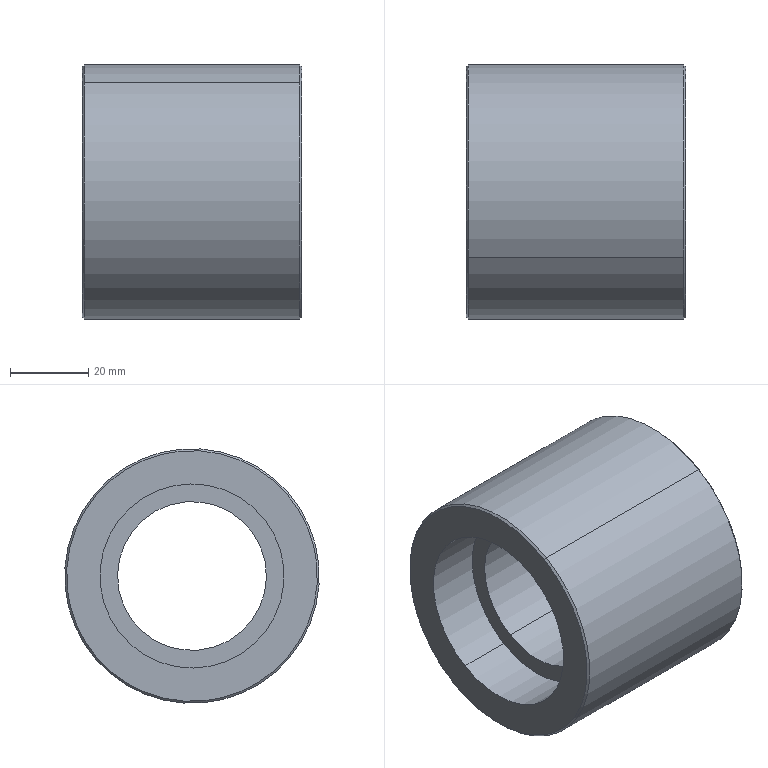Component | SolidWorks | PressHeadBearingHousing-1 | 1 solid | 36 faces | box 56 x 65 x 65 mm | volume 103574 mm3 | cylinder 20 | plane 10 | cone 6 | commonest cylinder face diameters 4.2 x12 47 x4 65 x2 38 x2
STEP:
#1=COLOUR_RGB('',0.7922,0.8196,0.9333);
#2=FILL_AREA_STYLE_COLOUR('',#1);
#3=FILL_AREA_STYLE('',(#2));
#4=SURFACE_STYLE_FILL_AREA(#3);
#5=SURFACE_SIDE_STYLE('',(#4));
#6=SURFACE_STYLE_USAGE(.BOTH.,#5);
#7=PRESENTATION_STYLE_ASSIGNMENT((#6));
#8=CARTESIAN_POINT('',(16.809,50.693,27.845));
#9=VERTEX_POINT('',#8);
#10=CARTESIAN_POINT('',(16.809,51.646,26.259));
#11=VERTEX_POINT('',#10);
#12=CARTESIAN_POINT('',(16.809,51.17,27.052));
#13=DIRECTION('',(-1.,-0.,-0.));
#14=DIRECTION('',(-0.,0.515,-0.8572));
#15=AXIS2_PLACEMENT_3D('',#12,#13,#14);
#16=CIRCLE('',#15,0.9252);
#17=EDGE_CURVE('',#9,#11,#16,.T.);
#18=ORIENTED_EDGE('',*,*,#17,.F.);
#19=CARTESIAN_POINT('',(16.257,50.693,27.845));
#20=VERTEX_POINT('',#19);
#21=CARTESIAN_POINT('',(16.809,50.693,27.845));
#22=DIRECTION('',(-1.,-0.,-0.));
#23=VECTOR('',#22,39.37);
#24=LINE('',#21,#23);
#25=EDGE_CURVE('',#9,#20,#24,.T.);
#26=ORIENTED_EDGE('',*,*,#25,.T.);
#27=CARTESIAN_POINT('',(16.257,51.646,26.259));
#28=VERTEX_POINT('',#27);
#29=CARTESIAN_POINT('',(16.257,51.17,27.052));
#30=DIRECTION('',(-1.,-0.,-0.));
#31=DIRECTION('',(-0.,0.515,-0.8572));
#32=AXIS2_PLACEMENT_3D('',#29,#30,#31);
#33=CIRCLE('',#32,0.9252);
#34=EDGE_CURVE('',#20,#28,#33,.T.);
#35=ORIENTED_EDGE('',*,*,#34,.T.);
#36=CARTESIAN_POINT('',(16.809,51.646,26.259));
#37=DIRECTION('',(-1.,-0.,-0.));
#38=VECTOR('',#37,39.37);
#39=LINE('',#36,#38);
#40=EDGE_CURVE('',#11,#28,#39,.T.);
#41=ORIENTED_EDGE('',*,*,#40,.F.);
#42=EDGE_LOOP('',(#18,#26,#35,#41));
#43=FACE_OUTER_BOUND('',#42,.T.);
#44=CARTESIAN_POINT('',(16.809,51.17,27.052));
#45=DIRECTION('',(-1.,-0.,-0.));
#46=DIRECTION('',(-0.,0.515,-0.8572));
#47=AXIS2_PLACEMENT_3D('',#44,#45,#46);
#48=CYLINDRICAL_SURFACE('',#47,0.9252);
#49=ADVANCED_FACE('',(#43),#48,.F.);
#50=CARTESIAN_POINT('',(17.872,51.231,25.879));
#51=VERTEX_POINT('',#50);
#52=CARTESIAN_POINT('',(17.872,51.146,26.02));
#53=VERTEX_POINT('',#52);
#54=CARTESIAN_POINT('',(17.872,51.189,25.95));
#55=DIRECTION('',(1.,0.,0.));
#56=DIRECTION('',(0.,-0.515,0.8572));
#57=AXIS2_PLACEMENT_3D('',#54,#55,#56);
#58=CIRCLE('',#57,0.08268);
#59=EDGE_CURVE('',#51,#53,#58,.T.);
#60=ORIENTED_EDGE('',*,*,#59,.F.);
#61=CARTESIAN_POINT('',(18.462,51.231,25.879));
#62=VERTEX_POINT('',#61);
#63=CARTESIAN_POINT('',(17.872,51.231,25.879));
#64=DIRECTION('',(1.,0.,0.));
#65=VECTOR('',#64,39.37);
#66=LINE('',#63,#65);
#67=EDGE_CURVE('',#51,#62,#66,.T.);
#68=ORIENTED_EDGE('',*,*,#67,.T.);
#69=CARTESIAN_POINT('',(18.462,51.146,26.02));
#70=VERTEX_POINT('',#69);
#71=CARTESIAN_POINT('',(18.462,51.189,25.95));
#72=DIRECTION('',(1.,0.,0.));
#73=DIRECTION('',(0.,-0.515,0.8572));
#74=AXIS2_PLACEMENT_3D('',#71,#72,#73);
#75=CIRCLE('',#74,0.08268);
#76=EDGE_CURVE('',#62,#70,#75,.T.);
#77=ORIENTED_EDGE('',*,*,#76,.T.);
#78=CARTESIAN_POINT('',(17.872,51.146,26.02));
#79=DIRECTION('',(1.,0.,0.));
#80=VECTOR('',#79,39.37);
#81=LINE('',#78,#80);
#82=EDGE_CURVE('',#53,#70,#81,.T.);
#83=ORIENTED_EDGE('',*,*,#82,.F.);
#84=EDGE_LOOP('',(#60,#68,#77,#83));
#85=FACE_OUTER_BOUND('',#84,.T.);
#86=CARTESIAN_POINT('',(17.872,51.189,25.95));
#87=DIRECTION('',(1.,0.,0.));
#88=DIRECTION('',(0.,-0.515,0.8572));
#89=AXIS2_PLACEMENT_3D('',#86,#87,#88);
#90=CYLINDRICAL_SURFACE('',#89,0.08268);
#91=ADVANCED_FACE('',(#85),#90,.F.);
#92=CARTESIAN_POINT('',(17.872,52.176,26.447));
#93=VERTEX_POINT('',#92);
#94=CARTESIAN_POINT('',(17.872,52.091,26.588));
#95=VERTEX_POINT('',#94);
#96=CARTESIAN_POINT('',(17.872,52.134,26.517));
#97=DIRECTION('',(1.,0.,0.));
#98=DIRECTION('',(0.,-0.515,0.8572));
#99=AXIS2_PLACEMENT_3D('',#96,#97,#98);
#100=CIRCLE('',#99,0.08268);
#101=EDGE_CURVE('',#93,#95,#100,.T.);
#102=ORIENTED_EDGE('',*,*,#101,.F.);
#103=CARTESIAN_POINT('',(18.462,52.176,26.447));
#104=VERTEX_POINT('',#103);
#105=CARTESIAN_POINT('',(17.872,52.176,26.447));
#106=DIRECTION('',(1.,0.,0.));
#107=VECTOR('',#106,39.37);
#108=LINE('',#105,#107);
#109=EDGE_CURVE('',#93,#104,#108,.T.);
#110=ORIENTED_EDGE('',*,*,#109,.T.);
#111=CARTESIAN_POINT('',(18.462,52.091,26.588));
#112=VERTEX_POINT('',#111);
#113=CARTESIAN_POINT('',(18.462,52.134,26.517));
#114=DIRECTION('',(1.,0.,0.));
#115=DIRECTION('',(0.,-0.515,0.8572));
#116=AXIS2_PLACEMENT_3D('',#113,#114,#115);
#117=CIRCLE('',#116,0.08268);
#118=EDGE_CURVE('',#104,#112,#117,.T.);
#119=ORIENTED_EDGE('',*,*,#118,.T.);
#120=CARTESIAN_POINT('',(17.872,52.091,26.588));
#121=DIRECTION('',(1.,0.,0.));
#122=VECTOR('',#121,39.37);
#123=LINE('',#120,#122);
#124=EDGE_CURVE('',#95,#112,#123,.T.);
#125=ORIENTED_EDGE('',*,*,#124,.F.);
#126=EDGE_LOOP('',(#102,#110,#119,#125));
#127=FACE_OUTER_BOUND('',#126,.T.);
#128=CARTESIAN_POINT('',(17.872,52.134,26.517));
#129=DIRECTION('',(1.,0.,0.));
#130=DIRECTION('',(0.,-0.515,0.8572));
#131=AXIS2_PLACEMENT_3D('',#128,#129,#130);
#132=CYLINDRICAL_SURFACE('',#131,0.08268);
#133=ADVANCED_FACE('',(#127),#132,.F.);
#134=CARTESIAN_POINT('',(17.872,52.157,27.549));
#135=VERTEX_POINT('',#134);
#136=CARTESIAN_POINT('',(17.872,52.072,27.69));
#137=VERTEX_POINT('',#136);
#138=CARTESIAN_POINT('',(17.872,52.114,27.62));
#139=DIRECTION('',(1.,0.,0.));
#140=DIRECTION('',(0.,-0.515,0.8572));
#141=AXIS2_PLACEMENT_3D('',#138,#139,#140);
#142=CIRCLE('',#141,0.08268);
#143=EDGE_CURVE('',#135,#137,#142,.T.);
#144=ORIENTED_EDGE('',*,*,#143,.F.);
#145=CARTESIAN_POINT('',(18.462,52.157,27.549));
#146=VERTEX_POINT('',#145);
#147=CARTESIAN_POINT('',(17.872,52.157,27.549));
#148=DIRECTION('',(1.,0.,0.));
#149=VECTOR('',#148,39.37);
#150=LINE('',#147,#149);
#151=EDGE_CURVE('',#135,#146,#150,.T.);
#152=ORIENTED_EDGE('',*,*,#151,.T.);
#153=CARTESIAN_POINT('',(18.462,52.072,27.69));
#154=VERTEX_POINT('',#153);
#155=CARTESIAN_POINT('',(18.462,52.114,27.62));
#156=DIRECTION('',(1.,0.,0.));
#157=DIRECTION('',(0.,-0.515,0.8572));
#158=AXIS2_PLACEMENT_3D('',#155,#156,#157);
#159=CIRCLE('',#158,0.08268);
#160=EDGE_CURVE('',#146,#154,#159,.T.);
#161=ORIENTED_EDGE('',*,*,#160,.T.);
#162=CARTESIAN_POINT('',(17.872,52.072,27.69));
#163=DIRECTION('',(1.,0.,0.));
#164=VECTOR('',#163,39.37);
#165=LINE('',#162,#164);
#166=EDGE_CURVE('',#137,#154,#165,.T.);
#167=ORIENTED_EDGE('',*,*,#166,.F.);
#168=EDGE_LOOP('',(#144,#152,#161,#167));
#169=FACE_OUTER_BOUND('',#168,.T.);
#170=CARTESIAN_POINT('',(17.872,52.114,27.62));
#171=DIRECTION('',(1.,0.,0.));
#172=DIRECTION('',(0.,-0.515,0.8572));
#173=AXIS2_PLACEMENT_3D('',#170,#171,#172);
#174=CYLINDRICAL_SURFACE('',#173,0.08268);
#175=ADVANCED_FACE('',(#169),#174,.F.);
#176=CARTESIAN_POINT('',(17.872,51.193,28.083));
#177=VERTEX_POINT('',#176);
#178=CARTESIAN_POINT('',(17.872,51.108,28.225));
#179=VERTEX_POINT('',#178);
#180=CARTESIAN_POINT('',(17.872,51.15,28.154));
#181=DIRECTION('',(1.,0.,0.));
#182=DIRECTION('',(0.,-0.515,0.8572));
#183=AXIS2_PLACEMENT_3D('',#180,#181,#182);
#184=CIRCLE('',#183,0.08268);
#185=EDGE_CURVE('',#177,#179,#184,.T.);
#186=ORIENTED_EDGE('',*,*,#185,.F.);
#187=CARTESIAN_POINT('',(18.462,51.193,28.083));
#188=VERTEX_POINT('',#187);
#189=CARTESIAN_POINT('',(17.872,51.193,28.083));
#190=DIRECTION('',(1.,0.,0.));
#191=VECTOR('',#190,39.37);
#192=LINE('',#189,#191);
#193=EDGE_CURVE('',#177,#188,#192,.T.);
#194=ORIENTED_EDGE('',*,*,#193,.T.);
#195=CARTESIAN_POINT('',(18.462,51.108,28.225));
#196=VERTEX_POINT('',#195);
#197=CARTESIAN_POINT('',(18.462,51.15,28.154));
#198=DIRECTION('',(1.,0.,0.));
#199=DIRECTION('',(0.,-0.515,0.8572));
#200=AXIS2_PLACEMENT_3D('',#197,#198,#199);
#201=CIRCLE('',#200,0.08268);
#202=EDGE_CURVE('',#188,#196,#201,.T.);
#203=ORIENTED_EDGE('',*,*,#202,.T.);
#204=CARTESIAN_POINT('',(17.872,51.108,28.225));
#205=DIRECTION('',(1.,0.,0.));
#206=VECTOR('',#205,39.37);
#207=LINE('',#204,#206);
#208=EDGE_CURVE('',#179,#196,#207,.T.);
#209=ORIENTED_EDGE('',*,*,#208,.F.);
#210=EDGE_LOOP('',(#186,#194,#203,#209));
#211=FACE_OUTER_BOUND('',#210,.T.);
#212=CARTESIAN_POINT('',(17.872,51.15,28.154));
#213=DIRECTION('',(1.,0.,0.));
#214=DIRECTION('',(0.,-0.515,0.8572));
#215=AXIS2_PLACEMENT_3D('',#212,#213,#214);
#216=CYLINDRICAL_SURFACE('',#215,0.08268);
#217=ADVANCED_FACE('',(#211),#216,.F.);
#218=CARTESIAN_POINT('',(17.872,50.267,26.413));
#219=VERTEX_POINT('',#218);
#220=CARTESIAN_POINT('',(17.872,50.182,26.555));
#221=VERTEX_POINT('',#220);
#222=CARTESIAN_POINT('',(17.872,50.225,26.484));
#223=DIRECTION('',(1.,0.,0.));
#224=DIRECTION('',(0.,-0.515,0.8572));
#225=AXIS2_PLACEMENT_3D('',#222,#223,#224);
#226=CIRCLE('',#225,0.08268);
#227=EDGE_CURVE('',#219,#221,#226,.T.);
#228=ORIENTED_EDGE('',*,*,#227,.F.);
#229=CARTESIAN_POINT('',(18.462,50.267,26.413));
#230=VERTEX_POINT('',#229);
#231=CARTESIAN_POINT('',(17.872,50.267,26.413));
#232=DIRECTION('',(1.,0.,0.));
#233=VECTOR('',#232,39.37);
#234=LINE('',#231,#233);
#235=EDGE_CURVE('',#219,#230,#234,.T.);
#236=ORIENTED_EDGE('',*,*,#235,.T.);
#237=CARTESIAN_POINT('',(18.462,50.182,26.555));
#238=VERTEX_POINT('',#237);
#239=CARTESIAN_POINT('',(18.462,50.225,26.484));
#240=DIRECTION('',(1.,0.,0.));
#241=DIRECTION('',(0.,-0.515,0.8572));
#242=AXIS2_PLACEMENT_3D('',#239,#240,#241);
#243=CIRCLE('',#242,0.08268);
#244=EDGE_CURVE('',#230,#238,#243,.T.);
#245=ORIENTED_EDGE('',*,*,#244,.T.);
#246=CARTESIAN_POINT('',(17.872,50.182,26.555));
#247=DIRECTION('',(1.,0.,0.));
#248=VECTOR('',#247,39.37);
#249=LINE('',#246,#248);
#250=EDGE_CURVE('',#221,#238,#249,.T.);
#251=ORIENTED_EDGE('',*,*,#250,.F.);
#252=EDGE_LOOP('',(#228,#236,#245,#251));
#253=FACE_OUTER_BOUND('',#252,.T.);
#254=CARTESIAN_POINT('',(17.872,50.225,26.484));
#255=DIRECTION('',(1.,0.,0.));
#256=DIRECTION('',(0.,-0.515,0.8572));
#257=AXIS2_PLACEMENT_3D('',#254,#255,#256);
#258=CYLINDRICAL_SURFACE('',#257,0.08268);
#259=ADVANCED_FACE('',(#253),#258,.F.);
#260=CARTESIAN_POINT('',(17.872,50.248,27.515));
#261=VERTEX_POINT('',#260);
#262=CARTESIAN_POINT('',(17.872,50.163,27.657));
#263=VERTEX_POINT('',#262);
#264=CARTESIAN_POINT('',(17.872,50.205,27.586));
#265=DIRECTION('',(1.,0.,0.));
#266=DIRECTION('',(0.,-0.515,0.8572));
#267=AXIS2_PLACEMENT_3D('',#264,#265,#266);
#268=CIRCLE('',#267,0.08268);
#269=EDGE_CURVE('',#261,#263,#268,.T.);
#270=ORIENTED_EDGE('',*,*,#269,.F.);
#271=CARTESIAN_POINT('',(18.462,50.248,27.515));
#272=VERTEX_POINT('',#271);
#273=CARTESIAN_POINT('',(17.872,50.248,27.515));
#274=DIRECTION('',(1.,0.,0.));
#275=VECTOR('',#274,39.37);
#276=LINE('',#273,#275);
#277=EDGE_CURVE('',#261,#272,#276,.T.);
#278=ORIENTED_EDGE('',*,*,#277,.T.);
#279=CARTESIAN_POINT('',(18.462,50.163,27.657));
#280=VERTEX_POINT('',#279);
#281=CARTESIAN_POINT('',(18.462,50.205,27.586));
#282=DIRECTION('',(1.,0.,0.));
#283=DIRECTION('',(0.,-0.515,0.8572));
#284=AXIS2_PLACEMENT_3D('',#281,#282,#283);
#285=CIRCLE('',#284,0.08268);
#286=EDGE_CURVE('',#272,#280,#285,.T.);
#287=ORIENTED_EDGE('',*,*,#286,.T.);
#288=CARTESIAN_POINT('',(17.872,50.163,27.657));
#289=DIRECTION('',(1.,0.,0.));
#290=VECTOR('',#289,39.37);
#291=LINE('',#288,#290);
#292=EDGE_CURVE('',#263,#280,#291,.T.);
#293=ORIENTED_EDGE('',*,*,#292,.F.);
#294=EDGE_LOOP('',(#270,#278,#287,#293));
#295=FACE_OUTER_BOUND('',#294,.T.);
#296=CARTESIAN_POINT('',(17.872,50.205,27.586));
#297=DIRECTION('',(1.,0.,0.));
#298=DIRECTION('',(0.,-0.515,0.8572));
#299=AXIS2_PLACEMENT_3D('',#296,#297,#298);
#300=CYLINDRICAL_SURFACE('',#299,0.08268);
#301=ADVANCED_FACE('',(#295),#300,.F.);
#302=CARTESIAN_POINT('',(18.442,51.646,26.259));
#303=VERTEX_POINT('',#302);
#304=CARTESIAN_POINT('',(18.442,50.693,27.845));
#305=VERTEX_POINT('',#304);
#306=CARTESIAN_POINT('',(18.442,51.17,27.052));
#307=DIRECTION('',(1.,0.,0.));
#308=DIRECTION('',(0.,-0.515,0.8572));
#309=AXIS2_PLACEMENT_3D('',#306,#307,#308);
#310=CIRCLE('',#309,0.9252);
#311=EDGE_CURVE('',#303,#305,#310,.T.);
#312=ORIENTED_EDGE('',*,*,#311,.F.);
#313=CARTESIAN_POINT('',(18.462,51.656,26.242));
#314=VERTEX_POINT('',#313);
#315=CARTESIAN_POINT('',(18.442,51.646,26.259));
#316=DIRECTION('',(0.7071,0.3642,-0.6061));
#317=VECTOR('',#316,39.37);
#318=LINE('',#315,#317);
#319=EDGE_CURVE('',#303,#314,#318,.T.);
#320=ORIENTED_EDGE('',*,*,#319,.T.);
#321=CARTESIAN_POINT('',(18.462,50.683,27.862));
#322=VERTEX_POINT('',#321);
#323=CARTESIAN_POINT('',(18.462,51.17,27.052));
#324=DIRECTION('',(-1.,-0.,-0.));
#325=DIRECTION('',(0.,-0.515,0.8572));
#326=AXIS2_PLACEMENT_3D('',#323,#324,#325);
#327=CIRCLE('',#326,0.9449);
#328=EDGE_CURVE('',#322,#314,#327,.T.);
#329=ORIENTED_EDGE('',*,*,#328,.F.);
#330=CARTESIAN_POINT('',(18.442,50.693,27.845));
#331=DIRECTION('',(0.7071,-0.3642,0.6061));
#332=VECTOR('',#331,39.37);
#333=LINE('',#330,#332);
#334=EDGE_CURVE('',#305,#322,#333,.T.);
#335=ORIENTED_EDGE('',*,*,#334,.F.);
#336=EDGE_LOOP('',(#312,#320,#329,#335));
#337=FACE_OUTER_BOUND('',#336,.T.);
#338=CARTESIAN_POINT('',(18.442,51.17,27.052));
#339=DIRECTION('',(1.,0.,0.));
#340=DIRECTION('',(0.,-0.515,0.8572));
#341=AXIS2_PLACEMENT_3D('',#338,#339,#340);
#342=CONICAL_SURFACE('',#341,0.9252,0.7854);
#343=ADVANCED_FACE('',(#337),#342,.F.);
#344=CARTESIAN_POINT('',(18.462,50.521,28.132));
#345=VERTEX_POINT('',#344);
#346=CARTESIAN_POINT('',(18.462,51.818,25.972));
#347=VERTEX_POINT('',#346);
#348=CARTESIAN_POINT('',(18.462,51.17,27.052));
#349=DIRECTION('',(1.,0.,0.));
#350=DIRECTION('',(0.,-0.515,0.8572));
#351=AXIS2_PLACEMENT_3D('',#348,#349,#350);
#352=CIRCLE('',#351,1.26);
#353=EDGE_CURVE('',#345,#347,#352,.T.);
#354=ORIENTED_EDGE('',*,*,#353,.F.);
#355=CARTESIAN_POINT('',(18.442,50.511,28.149));
#356=VERTEX_POINT('',#355);
#357=CARTESIAN_POINT('',(18.462,50.521,28.132));
#358=DIRECTION('',(-0.7071,-0.3642,0.6061));
#359=VECTOR('',#358,39.37);
#360=LINE('',#357,#359);
#361=EDGE_CURVE('',#345,#356,#360,.T.);
#362=ORIENTED_EDGE('',*,*,#361,.T.);
#363=CARTESIAN_POINT('',(18.442,51.829,25.955));
#364=VERTEX_POINT('',#363);
#365=CARTESIAN_POINT('',(18.442,51.17,27.052));
#366=DIRECTION('',(-1.,-0.,-0.));
#367=DIRECTION('',(0.,-0.515,0.8572));
#368=AXIS2_PLACEMENT_3D('',#365,#366,#367);
#369=CIRCLE('',#368,1.28);
#370=EDGE_CURVE('',#364,#356,#369,.T.);
#371=ORIENTED_EDGE('',*,*,#370,.F.);
#372=CARTESIAN_POINT('',(18.462,51.818,25.972));
#373=DIRECTION('',(-0.7071,0.3642,-0.6061));
#374=VECTOR('',#373,39.37);
#375=LINE('',#372,#374);
#376=EDGE_CURVE('',#347,#364,#375,.T.);
#377=ORIENTED_EDGE('',*,*,#376,.F.);
#378=EDGE_LOOP('',(#354,#362,#371,#377));
#379=FACE_OUTER_BOUND('',#378,.T.);
#380=CARTESIAN_POINT('',(18.462,51.17,27.052));
#381=DIRECTION('',(-1.,-0.,-0.));
#382=DIRECTION('',(-0.,0.515,-0.8572));
#383=AXIS2_PLACEMENT_3D('',#380,#381,#382);
#384=CONICAL_SURFACE('',#383,1.26,0.7854);
#385=ADVANCED_FACE('',(#379),#384,.T.);
#386=CARTESIAN_POINT('',(16.257,51.818,25.972));
#387=VERTEX_POINT('',#386);
#388=CARTESIAN_POINT('',(16.257,50.521,28.132));
#389=VERTEX_POINT('',#388);
#390=CARTESIAN_POINT('',(16.257,51.17,27.052));
#391=DIRECTION('',(-1.,-0.,-0.));
#392=DIRECTION('',(0.,-0.515,0.8572));
#393=AXIS2_PLACEMENT_3D('',#390,#391,#392);
#394=CIRCLE('',#393,1.26);
#395=EDGE_CURVE('',#387,#389,#394,.T.);
#396=ORIENTED_EDGE('',*,*,#395,.F.);
#397=CARTESIAN_POINT('',(16.277,51.829,25.955));
#398=VERTEX_POINT('',#397);
#399=CARTESIAN_POINT('',(16.277,51.829,25.955));
#400=DIRECTION('',(0.7071,0.3642,-0.6061));
#401=VECTOR('',#400,39.37);
#402=LINE('',#399,#401);
#403=EDGE_CURVE('',#387,#398,#402,.T.);
#404=ORIENTED_EDGE('',*,*,#403,.T.);
#405=CARTESIAN_POINT('',(16.277,50.511,28.149));
#406=VERTEX_POINT('',#405);
#407=CARTESIAN_POINT('',(16.277,51.17,27.052));
#408=DIRECTION('',(1.,0.,0.));
#409=DIRECTION('',(0.,-0.515,0.8572));
#410=AXIS2_PLACEMENT_3D('',#407,#408,#409);
#411=CIRCLE('',#410,1.28);
#412=EDGE_CURVE('',#406,#398,#411,.T.);
#413=ORIENTED_EDGE('',*,*,#412,.F.);
#414=CARTESIAN_POINT('',(16.277,50.511,28.149));
#415=DIRECTION('',(0.7071,-0.3642,0.6061));
#416=VECTOR('',#415,39.37);
#417=LINE('',#414,#416);
#418=EDGE_CURVE('',#389,#406,#417,.T.);
#419=ORIENTED_EDGE('',*,*,#418,.F.);
#420=EDGE_LOOP('',(#396,#404,#413,#419));
#421=FACE_OUTER_BOUND('',#420,.T.);
#422=CARTESIAN_POINT('',(16.277,51.17,27.052));
#423=DIRECTION('',(1.,0.,0.));
#424=DIRECTION('',(0.,-0.515,0.8572));
#425=AXIS2_PLACEMENT_3D('',#422,#423,#424);
#426=CONICAL_SURFACE('',#425,1.28,0.7854);
#427=ADVANCED_FACE('',(#421),#426,.T.);
#428=CARTESIAN_POINT('',(17.872,51.646,26.259));
#429=VERTEX_POINT('',#428);
#430=CARTESIAN_POINT('',(17.872,50.693,27.845));
#431=VERTEX_POINT('',#430);
#432=CARTESIAN_POINT('',(17.872,51.17,27.052));
#433=DIRECTION('',(1.,0.,0.));
#434=DIRECTION('',(0.,-0.515,0.8572));
#435=AXIS2_PLACEMENT_3D('',#432,#433,#434);
#436=CIRCLE('',#435,0.9252);
#437=EDGE_CURVE('',#429,#431,#436,.T.);
#438=ORIENTED_EDGE('',*,*,#437,.F.);
#439=CARTESIAN_POINT('',(17.872,51.646,26.259));
#440=DIRECTION('',(1.,0.,0.));
#441=VECTOR('',#440,39.37);
#442=LINE('',#439,#441);
#443=EDGE_CURVE('',#429,#303,#442,.T.);
#444=ORIENTED_EDGE('',*,*,#443,.T.);
#445=ORIENTED_EDGE('',*,*,#311,.T.);
#446=CARTESIAN_POINT('',(17.872,50.693,27.845));
#447=DIRECTION('',(1.,0.,0.));
#448=VECTOR('',#447,39.37);
#449=LINE('',#446,#448);
#450=EDGE_CURVE('',#431,#305,#449,.T.);
#451=ORIENTED_EDGE('',*,*,#450,.F.);
#452=EDGE_LOOP('',(#438,#444,#445,#451));
#453=FACE_OUTER_BOUND('',#452,.T.);
#454=CARTESIAN_POINT('',(17.872,51.17,27.052));
#455=DIRECTION('',(1.,0.,0.));
#456=DIRECTION('',(0.,-0.515,0.8572));
#457=AXIS2_PLACEMENT_3D('',#454,#455,#456);
#458=CYLINDRICAL_SURFACE('',#457,0.9252);
#459=ADVANCED_FACE('',(#453),#458,.F.);
#460=ORIENTED_EDGE('',*,*,#370,.T.);
#461=CARTESIAN_POINT('',(17.045,50.511,28.149));
#462=DIRECTION('',(-1.,-0.,-0.));
#463=VECTOR('',#462,39.37);
#464=LINE('',#461,#463);
#465=EDGE_CURVE('',#356,#406,#464,.T.);
#466=ORIENTED_EDGE('',*,*,#465,.T.);
#467=ORIENTED_EDGE('',*,*,#412,.T.);
#468=CARTESIAN_POINT('',(17.045,51.829,25.955));
#469=DIRECTION('',(-1.,-0.,-0.));
#470=VECTOR('',#469,39.37);
#471=LINE('',#468,#470);
#472=EDGE_CURVE('',#364,#398,#471,.T.);
#473=ORIENTED_EDGE('',*,*,#472,.F.);
#474=EDGE_LOOP('',(#460,#466,#467,#473));
#475=FACE_OUTER_BOUND('',#474,.T.);
#476=CARTESIAN_POINT('',(17.045,51.17,27.052));
#477=DIRECTION('',(-1.,-0.,-0.));
#478=DIRECTION('',(-0.,0.515,-0.8572));
#479=AXIS2_PLACEMENT_3D('',#476,#477,#478);
#480=CYLINDRICAL_SURFACE('',#479,1.28);
#481=ADVANCED_FACE('',(#475),#480,.T.);
#482=CARTESIAN_POINT('',(16.809,51.555,26.411));
#483=VERTEX_POINT('',#482);
#484=CARTESIAN_POINT('',(16.809,50.784,27.693));
#485=VERTEX_POINT('',#484);
#486=CARTESIAN_POINT('',(16.809,51.17,27.052));
#487=DIRECTION('',(1.,0.,0.));
#488=DIRECTION('',(-0.,0.515,-0.8572));
#489=AXIS2_PLACEMENT_3D('',#486,#487,#488);
#490=CIRCLE('',#489,0.748);
#491=EDGE_CURVE('',#483,#485,#490,.T.);
#492=ORIENTED_EDGE('',*,*,#491,.F.);
#493=CARTESIAN_POINT('',(17.872,51.555,26.411));
#494=VERTEX_POINT('',#493);
#495=CARTESIAN_POINT('',(16.257,51.555,26.411));
#496=DIRECTION('',(1.,0.,0.));
#497=VECTOR('',#496,39.37);
#498=LINE('',#495,#497);
#499=EDGE_CURVE('',#483,#494,#498,.T.);
#500=ORIENTED_EDGE('',*,*,#499,.T.);
#501=CARTESIAN_POINT('',(17.872,50.784,27.693));
#502=VERTEX_POINT('',#501);
#503=CARTESIAN_POINT('',(17.872,51.17,27.052));
#504=DIRECTION('',(1.,0.,0.));
#505=DIRECTION('',(0.,-0.515,0.8572));
#506=AXIS2_PLACEMENT_3D('',#503,#504,#505);
#507=CIRCLE('',#506,0.748);
#508=EDGE_CURVE('',#494,#502,#507,.T.);
#509=ORIENTED_EDGE('',*,*,#508,.T.);
#510=CARTESIAN_POINT('',(16.257,50.784,27.693));
#511=DIRECTION('',(1.,0.,0.));
#512=VECTOR('',#511,39.37);
#513=LINE('',#510,#512);
#514=EDGE_CURVE('',#485,#502,#513,.T.);
#515=ORIENTED_EDGE('',*,*,#514,.F.);
#516=EDGE_LOOP('',(#492,#500,#509,#515));
#517=FACE_OUTER_BOUND('',#516,.T.);
#518=CARTESIAN_POINT('',(16.257,51.17,27.052));
#519=DIRECTION('',(1.,0.,0.));
#520=DIRECTION('',(0.,-0.515,0.8572));
#521=AXIS2_PLACEMENT_3D('',#518,#519,#520);
#522=CYLINDRICAL_SURFACE('',#521,0.748);
#523=ADVANCED_FACE('',(#517),#522,.F.);
#524=ORIENTED_EDGE('',*,*,#499,.F.);
#525=CARTESIAN_POINT('',(16.809,51.17,27.052));
#526=DIRECTION('',(1.,0.,0.));
#527=DIRECTION('',(-0.,0.515,-0.8572));
#528=AXIS2_PLACEMENT_3D('',#525,#526,#527);
#529=CIRCLE('',#528,0.748);
#530=EDGE_CURVE('',#485,#483,#529,.T.);
#531=ORIENTED_EDGE('',*,*,#530,.F.);
#532=ORIENTED_EDGE('',*,*,#514,.T.);
#533=CARTESIAN_POINT('',(17.872,51.17,27.052));
#534=DIRECTION('',(1.,0.,0.));
#535=DIRECTION('',(0.,-0.515,0.8572));
#536=AXIS2_PLACEMENT_3D('',#533,#534,#535);
#537=CIRCLE('',#536,0.748);
#538=EDGE_CURVE('',#502,#494,#537,.T.);
#539=ORIENTED_EDGE('',*,*,#538,.T.);
#540=EDGE_LOOP('',(#524,#531,#532,#539));
#541=FACE_OUTER_BOUND('',#540,.T.);
#542=CARTESIAN_POINT('',(16.257,51.17,27.052));
#543=DIRECTION('',(1.,0.,0.));
#544=DIRECTION('',(0.,-0.515,0.8572));
#545=AXIS2_PLACEMENT_3D('',#542,#543,#544);
#546=CYLINDRICAL_SURFACE('',#545,0.748);
#547=ADVANCED_FACE('',(#541),#546,.F.);
#548=ORIENTED_EDGE('',*,*,#465,.F.);
#549=CARTESIAN_POINT('',(18.442,51.17,27.052));
#550=DIRECTION('',(-1.,-0.,-0.));
#551=DIRECTION('',(0.,-0.515,0.8572));
#552=AXIS2_PLACEMENT_3D('',#549,#550,#551);
#553=CIRCLE('',#552,1.28);
#554=EDGE_CURVE('',#356,#364,#553,.T.);
#555=ORIENTED_EDGE('',*,*,#554,.T.);
#556=ORIENTED_EDGE('',*,*,#472,.T.);
#557=CARTESIAN_POINT('',(16.277,51.17,27.052));
#558=DIRECTION('',(1.,0.,0.));
#559=DIRECTION('',(0.,-0.515,0.8572));
#560=AXIS2_PLACEMENT_3D('',#557,#558,#559);
#561=CIRCLE('',#560,1.28);
#562=EDGE_CURVE('',#398,#406,#561,.T.);
#563=ORIENTED_EDGE('',*,*,#562,.T.);
#564=EDGE_LOOP('',(#548,#555,#556,#563));
#565=FACE_OUTER_BOUND('',#564,.T.);
#566=CARTESIAN_POINT('',(17.045,51.17,27.052));
#567=DIRECTION('',(-1.,-0.,-0.));
#568=DIRECTION('',(-0.,0.515,-0.8572));
#569=AXIS2_PLACEMENT_3D('',#566,#567,#568);
#570=CYLINDRICAL_SURFACE('',#569,1.28);
#571=ADVANCED_FACE('',(#565),#570,.T.);
#572=CARTESIAN_POINT('',(16.257,51.17,27.052));
#573=DIRECTION('',(-1.,-0.,-0.));
#574=DIRECTION('',(-0.,0.515,-0.8572));
#575=AXIS2_PLACEMENT_3D('',#572,#573,#574);
#576=CIRCLE('',#575,0.9252);
#577=EDGE_CURVE('',#28,#20,#576,.T.);
#578=ORIENTED_EDGE('',*,*,#577,.F.);
#579=ORIENTED_EDGE('',*,*,#34,.F.);
#580=EDGE_LOOP('',(#578,#579));
#581=FACE_BOUND('',#580,.T.);
#582=CARTESIAN_POINT('',(16.257,51.17,27.052));
#583=DIRECTION('',(-1.,-0.,-0.));
#584=DIRECTION('',(0.,-0.515,0.8572));
#585=AXIS2_PLACEMENT_3D('',#582,#583,#584);
#586=CIRCLE('',#585,1.26);
#587=EDGE_CURVE('',#389,#387,#586,.T.);
#588=ORIENTED_EDGE('',*,*,#587,.T.);
#589=ORIENTED_EDGE('',*,*,#395,.T.);
#590=EDGE_LOOP('',(#588,#589));
#591=FACE_OUTER_BOUND('',#590,.T.);
#592=CARTESIAN_POINT('',(16.257,51.17,27.052));
#593=DIRECTION('',(1.,0.,0.));
#594=DIRECTION('',(0.,-0.515,0.8572));
#595=AXIS2_PLACEMENT_3D('',#592,#593,#594);
#596=PLANE('',#595);
#597=ADVANCED_FACE('',(#581,#591),#596,.F.);
#598=CARTESIAN_POINT('',(18.462,51.189,25.95));
#599=DIRECTION('',(1.,0.,0.));
#600=DIRECTION('',(0.,-0.515,0.8572));
#601=AXIS2_PLACEMENT_3D('',#598,#599,#600);
#602=CIRCLE('',#601,0.08268);
#603=EDGE_CURVE('',#70,#62,#602,.T.);
#604=ORIENTED_EDGE('',*,*,#603,.F.);
#605=ORIENTED_EDGE('',*,*,#76,.F.);
#606=EDGE_LOOP('',(#604,#605));
#607=FACE_BOUND('',#606,.T.);
#608=CARTESIAN_POINT('',(18.462,52.134,26.517));
#609=DIRECTION('',(1.,0.,0.));
#610=DIRECTION('',(0.,-0.515,0.8572));
#611=AXIS2_PLACEMENT_3D('',#608,#609,#610);
#612=CIRCLE('',#611,0.08268);
#613=EDGE_CURVE('',#112,#104,#612,.T.);
#614=ORIENTED_EDGE('',*,*,#613,.F.);
#615=ORIENTED_EDGE('',*,*,#118,.F.);
#616=EDGE_LOOP('',(#614,#615));
#617=FACE_BOUND('',#616,.T.);
#618=CARTESIAN_POINT('',(18.462,52.114,27.62));
#619=DIRECTION('',(1.,0.,0.));
#620=DIRECTION('',(0.,-0.515,0.8572));
#621=AXIS2_PLACEMENT_3D('',#618,#619,#620);
#622=CIRCLE('',#621,0.08268);
#623=EDGE_CURVE('',#154,#146,#622,.T.);
#624=ORIENTED_EDGE('',*,*,#623,.F.);
#625=ORIENTED_EDGE('',*,*,#160,.F.);
#626=EDGE_LOOP('',(#624,#625));
#627=FACE_BOUND('',#626,.T.);
#628=CARTESIAN_POINT('',(18.462,51.15,28.154));
#629=DIRECTION('',(1.,0.,0.));
#630=DIRECTION('',(0.,-0.515,0.8572));
#631=AXIS2_PLACEMENT_3D('',#628,#629,#630);
#632=CIRCLE('',#631,0.08268);
#633=EDGE_CURVE('',#196,#188,#632,.T.);
#634=ORIENTED_EDGE('',*,*,#633,.F.);
#635=ORIENTED_EDGE('',*,*,#202,.F.);
#636=EDGE_LOOP('',(#634,#635));
#637=FACE_BOUND('',#636,.T.);
#638=CARTESIAN_POINT('',(18.462,50.225,26.484));
#639=DIRECTION('',(1.,0.,0.));
#640=DIRECTION('',(0.,-0.515,0.8572));
#641=AXIS2_PLACEMENT_3D('',#638,#639,#640);
#642=CIRCLE('',#641,0.08268);
#643=EDGE_CURVE('',#238,#230,#642,.T.);
#644=ORIENTED_EDGE('',*,*,#643,.F.);
#645=ORIENTED_EDGE('',*,*,#244,.F.);
#646=EDGE_LOOP('',(#644,#645));
#647=FACE_BOUND('',#646,.T.);
#648=CARTESIAN_POINT('',(18.462,50.205,27.586));
#649=DIRECTION('',(1.,0.,0.));
#650=DIRECTION('',(0.,-0.515,0.8572));
#651=AXIS2_PLACEMENT_3D('',#648,#649,#650);
#652=CIRCLE('',#651,0.08268);
#653=EDGE_CURVE('',#280,#272,#652,.T.);
#654=ORIENTED_EDGE('',*,*,#653,.F.);
#655=ORIENTED_EDGE('',*,*,#286,.F.);
#656=EDGE_LOOP('',(#654,#655));
#657=FACE_BOUND('',#656,.T.);
#658=CARTESIAN_POINT('',(18.462,51.17,27.052));
#659=DIRECTION('',(1.,0.,0.));
#660=DIRECTION('',(0.,-0.515,0.8572));
#661=AXIS2_PLACEMENT_3D('',#658,#659,#660);
#662=CIRCLE('',#661,1.26);
#663=EDGE_CURVE('',#347,#345,#662,.T.);
#664=ORIENTED_EDGE('',*,*,#663,.T.);
#665=ORIENTED_EDGE('',*,*,#353,.T.);
#666=EDGE_LOOP('',(#664,#665));
#667=FACE_OUTER_BOUND('',#666,.T.);
#668=ORIENTED_EDGE('',*,*,#328,.T.);
#669=CARTESIAN_POINT('',(18.462,51.17,27.052));
#670=DIRECTION('',(-1.,-0.,-0.));
#671=DIRECTION('',(0.,-0.515,0.8572));
#672=AXIS2_PLACEMENT_3D('',#669,#670,#671);
#673=CIRCLE('',#672,0.9449);
#674=EDGE_CURVE('',#314,#322,#673,.T.);
#675=ORIENTED_EDGE('',*,*,#674,.T.);
#676=EDGE_LOOP('',(#668,#675));
#677=FACE_BOUND('',#676,.T.);
#678=CARTESIAN_POINT('',(18.462,51.17,27.052));
#679=DIRECTION('',(1.,0.,0.));
#680=DIRECTION('',(0.,-0.515,0.8572));
#681=AXIS2_PLACEMENT_3D('',#678,#679,#680);
#682=PLANE('',#681);
#683=ADVANCED_FACE('',(#607,#617,#627,#637,#647,#657,#667,#677),#682,.T.);
#684=ORIENTED_EDGE('',*,*,#443,.F.);
#685=CARTESIAN_POINT('',(17.872,51.17,27.052));
#686=DIRECTION('',(1.,0.,0.));
#687=DIRECTION('',(0.,-0.515,0.8572));
#688=AXIS2_PLACEMENT_3D('',#685,#686,#687);
#689=CIRCLE('',#688,0.9252);
#690=EDGE_CURVE('',#431,#429,#689,.T.);
#691=ORIENTED_EDGE('',*,*,#690,.F.);
#692=ORIENTED_EDGE('',*,*,#450,.T.);
#693=CARTESIAN_POINT('',(18.442,51.17,27.052));
#694=DIRECTION('',(1.,0.,0.));
#695=DIRECTION('',(0.,-0.515,0.8572));
#696=AXIS2_PLACEMENT_3D('',#693,#694,#695);
#697=CIRCLE('',#696,0.9252);
#698=EDGE_CURVE('',#305,#303,#697,.T.);
#699=ORIENTED_EDGE('',*,*,#698,.T.);
#700=EDGE_LOOP('',(#684,#691,#692,#699));
#701=FACE_OUTER_BOUND('',#700,.T.);
#702=CARTESIAN_POINT('',(17.872,51.17,27.052));
#703=DIRECTION('',(1.,0.,0.));
#704=DIRECTION('',(0.,-0.515,0.8572));
#705=AXIS2_PLACEMENT_3D('',#702,#703,#704);
#706=CYLINDRICAL_SURFACE('',#705,0.9252);
#707=ADVANCED_FACE('',(#701),#706,.F.);
#708=ORIENTED_EDGE('',*,*,#538,.F.);
#709=ORIENTED_EDGE('',*,*,#508,.F.);
#710=EDGE_LOOP('',(#708,#709));
#711=FACE_BOUND('',#710,.T.);
#712=ORIENTED_EDGE('',*,*,#690,.T.);
#713=ORIENTED_EDGE('',*,*,#437,.T.);
#714=EDGE_LOOP('',(#712,#713));
#715=FACE_OUTER_BOUND('',#714,.T.);
#716=CARTESIAN_POINT('',(17.872,51.17,27.052));
#717=DIRECTION('',(1.,0.,0.));
#718=DIRECTION('',(0.,-0.515,0.8572));
#719=AXIS2_PLACEMENT_3D('',#716,#717,#718);
#720=PLANE('',#719);
#721=ADVANCED_FACE('',(#711,#715),#720,.T.);
#722=ORIENTED_EDGE('',*,*,#403,.F.);
#723=ORIENTED_EDGE('',*,*,#587,.F.);
#724=ORIENTED_EDGE('',*,*,#418,.T.);
#725=ORIENTED_EDGE('',*,*,#562,.F.);
#726=EDGE_LOOP('',(#722,#723,#724,#725));
#727=FACE_OUTER_BOUND('',#726,.T.);
#728=CARTESIAN_POINT('',(16.277,51.17,27.052));
#729=DIRECTION('',(1.,0.,0.));
#730=DIRECTION('',(0.,-0.515,0.8572));
#731=AXIS2_PLACEMENT_3D('',#728,#729,#730);
#732=CONICAL_SURFACE('',#731,1.28,0.7854);
#733=ADVANCED_FACE('',(#727),#732,.T.);
#734=ORIENTED_EDGE('',*,*,#361,.F.);
#735=ORIENTED_EDGE('',*,*,#663,.F.);
#736=ORIENTED_EDGE('',*,*,#376,.T.);
#737=ORIENTED_EDGE('',*,*,#554,.F.);
#738=EDGE_LOOP('',(#734,#735,#736,#737));
#739=FACE_OUTER_BOUND('',#738,.T.);
#740=CARTESIAN_POINT('',(18.462,51.17,27.052));
#741=DIRECTION('',(-1.,-0.,-0.));
#742=DIRECTION('',(-0.,0.515,-0.8572));
#743=AXIS2_PLACEMENT_3D('',#740,#741,#742);
#744=CONICAL_SURFACE('',#743,1.26,0.7854);
#745=ADVANCED_FACE('',(#739),#744,.T.);
#746=ORIENTED_EDGE('',*,*,#319,.F.);
#747=ORIENTED_EDGE('',*,*,#698,.F.);
#748=ORIENTED_EDGE('',*,*,#334,.T.);
#749=ORIENTED_EDGE('',*,*,#674,.F.);
#750=EDGE_LOOP('',(#746,#747,#748,#749));
#751=FACE_OUTER_BOUND('',#750,.T.);
#752=CARTESIAN_POINT('',(18.442,51.17,27.052));
#753=DIRECTION('',(1.,0.,0.));
#754=DIRECTION('',(0.,-0.515,0.8572));
#755=AXIS2_PLACEMENT_3D('',#752,#753,#754);
#756=CONICAL_SURFACE('',#755,0.9252,0.7854);
#757=ADVANCED_FACE('',(#751),#756,.F.);
#758=ORIENTED_EDGE('',*,*,#277,.F.);
#759=CARTESIAN_POINT('',(17.872,50.205,27.586));
#760=DIRECTION('',(1.,0.,0.));
#761=DIRECTION('',(0.,-0.515,0.8572));
#762=AXIS2_PLACEMENT_3D('',#759,#760,#761);
#763=CIRCLE('',#762,0.08268);
#764=EDGE_CURVE('',#263,#261,#763,.T.);
#765=ORIENTED_EDGE('',*,*,#764,.F.);
#766=ORIENTED_EDGE('',*,*,#292,.T.);
#767=ORIENTED_EDGE('',*,*,#653,.T.);
#768=EDGE_LOOP('',(#758,#765,#766,#767));
#769=FACE_OUTER_BOUND('',#768,.T.);
#770=CARTESIAN_POINT('',(17.872,50.205,27.586));
#771=DIRECTION('',(1.,0.,0.));
#772=DIRECTION('',(0.,-0.515,0.8572));
#773=AXIS2_PLACEMENT_3D('',#770,#771,#772);
#774=CYLINDRICAL_SURFACE('',#773,0.08268);
#775=ADVANCED_FACE('',(#769),#774,.F.);
#776=ORIENTED_EDGE('',*,*,#764,.T.);
#777=ORIENTED_EDGE('',*,*,#269,.T.);
#778=EDGE_LOOP('',(#776,#777));
#779=FACE_OUTER_BOUND('',#778,.T.);
#780=CARTESIAN_POINT('',(17.872,50.205,27.586));
#781=DIRECTION('',(1.,0.,0.));
#782=DIRECTION('',(0.,-0.515,0.8572));
#783=AXIS2_PLACEMENT_3D('',#780,#781,#782);
#784=PLANE('',#783);
#785=ADVANCED_FACE('',(#779),#784,.T.);
#786=ORIENTED_EDGE('',*,*,#235,.F.);
#787=CARTESIAN_POINT('',(17.872,50.225,26.484));
#788=DIRECTION('',(1.,0.,0.));
#789=DIRECTION('',(0.,-0.515,0.8572));
#790=AXIS2_PLACEMENT_3D('',#787,#788,#789);
#791=CIRCLE('',#790,0.08268);
#792=EDGE_CURVE('',#221,#219,#791,.T.);
#793=ORIENTED_EDGE('',*,*,#792,.F.);
#794=ORIENTED_EDGE('',*,*,#250,.T.);
#795=ORIENTED_EDGE('',*,*,#643,.T.);
#796=EDGE_LOOP('',(#786,#793,#794,#795));
#797=FACE_OUTER_BOUND('',#796,.T.);
#798=CARTESIAN_POINT('',(17.872,50.225,26.484));
#799=DIRECTION('',(1.,0.,0.));
#800=DIRECTION('',(0.,-0.515,0.8572));
#801=AXIS2_PLACEMENT_3D('',#798,#799,#800);
#802=CYLINDRICAL_SURFACE('',#801,0.08268);
#803=ADVANCED_FACE('',(#797),#802,.F.);
#804=ORIENTED_EDGE('',*,*,#792,.T.);
#805=ORIENTED_EDGE('',*,*,#227,.T.);
#806=EDGE_LOOP('',(#804,#805));
#807=FACE_OUTER_BOUND('',#806,.T.);
#808=CARTESIAN_POINT('',(17.872,50.225,26.484));
#809=DIRECTION('',(1.,0.,0.));
#810=DIRECTION('',(0.,-0.515,0.8572));
#811=AXIS2_PLACEMENT_3D('',#808,#809,#810);
#812=PLANE('',#811);
#813=ADVANCED_FACE('',(#807),#812,.T.);
#814=ORIENTED_EDGE('',*,*,#193,.F.);
#815=CARTESIAN_POINT('',(17.872,51.15,28.154));
#816=DIRECTION('',(1.,0.,0.));
#817=DIRECTION('',(0.,-0.515,0.8572));
#818=AXIS2_PLACEMENT_3D('',#815,#816,#817);
#819=CIRCLE('',#818,0.08268);
#820=EDGE_CURVE('',#179,#177,#819,.T.);
#821=ORIENTED_EDGE('',*,*,#820,.F.);
#822=ORIENTED_EDGE('',*,*,#208,.T.);
#823=ORIENTED_EDGE('',*,*,#633,.T.);
#824=EDGE_LOOP('',(#814,#821,#822,#823));
#825=FACE_OUTER_BOUND('',#824,.T.);
#826=CARTESIAN_POINT('',(17.872,51.15,28.154));
#827=DIRECTION('',(1.,0.,0.));
#828=DIRECTION('',(0.,-0.515,0.8572));
#829=AXIS2_PLACEMENT_3D('',#826,#827,#828);
#830=CYLINDRICAL_SURFACE('',#829,0.08268);
#831=ADVANCED_FACE('',(#825),#830,.F.);
#832=ORIENTED_EDGE('',*,*,#820,.T.);
#833=ORIENTED_EDGE('',*,*,#185,.T.);
#834=EDGE_LOOP('',(#832,#833));
#835=FACE_OUTER_BOUND('',#834,.T.);
#836=CARTESIAN_POINT('',(17.872,51.15,28.154));
#837=DIRECTION('',(1.,0.,0.));
#838=DIRECTION('',(0.,-0.515,0.8572));
#839=AXIS2_PLACEMENT_3D('',#836,#837,#838);
#840=PLANE('',#839);
#841=ADVANCED_FACE('',(#835),#840,.T.);
#842=ORIENTED_EDGE('',*,*,#151,.F.);
#843=CARTESIAN_POINT('',(17.872,52.114,27.62));
#844=DIRECTION('',(1.,0.,0.));
#845=DIRECTION('',(0.,-0.515,0.8572));
#846=AXIS2_PLACEMENT_3D('',#843,#844,#845);
#847=CIRCLE('',#846,0.08268);
#848=EDGE_CURVE('',#137,#135,#847,.T.);
#849=ORIENTED_EDGE('',*,*,#848,.F.);
#850=ORIENTED_EDGE('',*,*,#166,.T.);
#851=ORIENTED_EDGE('',*,*,#623,.T.);
#852=EDGE_LOOP('',(#842,#849,#850,#851));
#853=FACE_OUTER_BOUND('',#852,.T.);
#854=CARTESIAN_POINT('',(17.872,52.114,27.62));
#855=DIRECTION('',(1.,0.,0.));
#856=DIRECTION('',(0.,-0.515,0.8572));
#857=AXIS2_PLACEMENT_3D('',#854,#855,#856);
#858=CYLINDRICAL_SURFACE('',#857,0.08268);
#859=ADVANCED_FACE('',(#853),#858,.F.);
#860=ORIENTED_EDGE('',*,*,#848,.T.);
#861=ORIENTED_EDGE('',*,*,#143,.T.);
#862=EDGE_LOOP('',(#860,#861));
#863=FACE_OUTER_BOUND('',#862,.T.);
#864=CARTESIAN_POINT('',(17.872,52.114,27.62));
#865=DIRECTION('',(1.,0.,0.));
#866=DIRECTION('',(0.,-0.515,0.8572));
#867=AXIS2_PLACEMENT_3D('',#864,#865,#866);
#868=PLANE('',#867);
#869=ADVANCED_FACE('',(#863),#868,.T.);
#870=ORIENTED_EDGE('',*,*,#109,.F.);
#871=CARTESIAN_POINT('',(17.872,52.134,26.517));
#872=DIRECTION('',(1.,0.,0.));
#873=DIRECTION('',(0.,-0.515,0.8572));
#874=AXIS2_PLACEMENT_3D('',#871,#872,#873);
#875=CIRCLE('',#874,0.08268);
#876=EDGE_CURVE('',#95,#93,#875,.T.);
#877=ORIENTED_EDGE('',*,*,#876,.F.);
#878=ORIENTED_EDGE('',*,*,#124,.T.);
#879=ORIENTED_EDGE('',*,*,#613,.T.);
#880=EDGE_LOOP('',(#870,#877,#878,#879));
#881=FACE_OUTER_BOUND('',#880,.T.);
#882=CARTESIAN_POINT('',(17.872,52.134,26.517));
#883=DIRECTION('',(1.,0.,0.));
#884=DIRECTION('',(0.,-0.515,0.8572));
#885=AXIS2_PLACEMENT_3D('',#882,#883,#884);
#886=CYLINDRICAL_SURFACE('',#885,0.08268);
#887=ADVANCED_FACE('',(#881),#886,.F.);
#888=ORIENTED_EDGE('',*,*,#876,.T.);
#889=ORIENTED_EDGE('',*,*,#101,.T.);
#890=EDGE_LOOP('',(#888,#889));
#891=FACE_OUTER_BOUND('',#890,.T.);
#892=CARTESIAN_POINT('',(17.872,52.134,26.517));
#893=DIRECTION('',(1.,0.,0.));
#894=DIRECTION('',(0.,-0.515,0.8572));
#895=AXIS2_PLACEMENT_3D('',#892,#893,#894);
#896=PLANE('',#895);
#897=ADVANCED_FACE('',(#891),#896,.T.);
#898=ORIENTED_EDGE('',*,*,#67,.F.);
#899=CARTESIAN_POINT('',(17.872,51.189,25.95));
#900=DIRECTION('',(1.,0.,0.));
#901=DIRECTION('',(0.,-0.515,0.8572));
#902=AXIS2_PLACEMENT_3D('',#899,#900,#901);
#903=CIRCLE('',#902,0.08268);
#904=EDGE_CURVE('',#53,#51,#903,.T.);
#905=ORIENTED_EDGE('',*,*,#904,.F.);
#906=ORIENTED_EDGE('',*,*,#82,.T.);
#907=ORIENTED_EDGE('',*,*,#603,.T.);
#908=EDGE_LOOP('',(#898,#905,#906,#907));
#909=FACE_OUTER_BOUND('',#908,.T.);
#910=CARTESIAN_POINT('',(17.872,51.189,25.95));
#911=DIRECTION('',(1.,0.,0.));
#912=DIRECTION('',(0.,-0.515,0.8572));
#913=AXIS2_PLACEMENT_3D('',#910,#911,#912);
#914=CYLINDRICAL_SURFACE('',#913,0.08268);
#915=ADVANCED_FACE('',(#909),#914,.F.);
#916=ORIENTED_EDGE('',*,*,#904,.T.);
#917=ORIENTED_EDGE('',*,*,#59,.T.);
#918=EDGE_LOOP('',(#916,#917));
#919=FACE_OUTER_BOUND('',#918,.T.);
#920=CARTESIAN_POINT('',(17.872,51.189,25.95));
#921=DIRECTION('',(1.,0.,0.));
#922=DIRECTION('',(0.,-0.515,0.8572));
#923=AXIS2_PLACEMENT_3D('',#920,#921,#922);
#924=PLANE('',#923);
#925=ADVANCED_FACE('',(#919),#924,.T.);
#926=CARTESIAN_POINT('',(16.809,51.17,27.052));
#927=DIRECTION('',(-1.,-0.,-0.));
#928=DIRECTION('',(-0.,0.515,-0.8572));
#929=AXIS2_PLACEMENT_3D('',#926,#927,#928);
#930=CIRCLE('',#929,0.9252);
#931=EDGE_CURVE('',#11,#9,#930,.T.);
#932=ORIENTED_EDGE('',*,*,#931,.T.);
#933=ORIENTED_EDGE('',*,*,#17,.T.);
#934=EDGE_LOOP('',(#932,#933));
#935=FACE_OUTER_BOUND('',#934,.T.);
#936=ORIENTED_EDGE('',*,*,#530,.T.);
#937=ORIENTED_EDGE('',*,*,#491,.T.);
#938=EDGE_LOOP('',(#936,#937));
#939=FACE_BOUND('',#938,.T.);
#940=CARTESIAN_POINT('',(16.809,51.17,27.052));
#941=DIRECTION('',(-1.,-0.,-0.));
#942=DIRECTION('',(-0.,0.515,-0.8572));
#943=AXIS2_PLACEMENT_3D('',#940,#941,#942);
#944=PLANE('',#943);
#945=ADVANCED_FACE('',(#935,#939),#944,.T.);
#946=ORIENTED_EDGE('',*,*,#25,.F.);
#947=ORIENTED_EDGE('',*,*,#931,.F.);
#948=ORIENTED_EDGE('',*,*,#40,.T.);
#949=ORIENTED_EDGE('',*,*,#577,.T.);
#950=EDGE_LOOP('',(#946,#947,#948,#949));
#951=FACE_OUTER_BOUND('',#950,.T.);
#952=CARTESIAN_POINT('',(16.809,51.17,27.052));
#953=DIRECTION('',(-1.,-0.,-0.));
#954=DIRECTION('',(-0.,0.515,-0.8572));
#955=AXIS2_PLACEMENT_3D('',#952,#953,#954);
#956=CYLINDRICAL_SURFACE('',#955,0.9252);
#957=ADVANCED_FACE('',(#951),#956,.F.);
#958=CLOSED_SHELL('',(#49,#91,#133,#175,#217,#259,#301,#343,#385,#427,#459,#481,#523,#547,#571,#597,#683,#707,#721,#733,#745,#757,#775,#785,#803,#813,#831,#841,#859,#869,#887,#897,#915,#925,#945,#957));
#959=MANIFOLD_SOLID_BREP('',#958);
#960=STYLED_ITEM('',(#7),#959);
#961=(LENGTH_UNIT()NAMED_UNIT(*)SI_UNIT($,.METRE.));
#962=LENGTH_MEASURE_WITH_UNIT(LENGTH_MEASURE(0.0254),#961);
#963=DIMENSIONAL_EXPONENTS(1.,0.,0.,0.,0.,0.,0.);
#964=(CONVERSION_BASED_UNIT('',#962)LENGTH_UNIT()NAMED_UNIT(#963));
#965=UNCERTAINTY_MEASURE_WITH_UNIT(LENGTH_MEASURE(0.00001),#964,'','');
#966=(NAMED_UNIT(*)PLANE_ANGLE_UNIT()SI_UNIT($,.RADIAN.));
#967=(NAMED_UNIT(*)SI_UNIT($,.STERADIAN.)SOLID_ANGLE_UNIT());
#968=(GEOMETRIC_REPRESENTATION_CONTEXT(3)GLOBAL_UNCERTAINTY_ASSIGNED_CONTEXT((#965))GLOBAL_UNIT_ASSIGNED_CONTEXT((#964,#966,#967))REPRESENTATION_CONTEXT('',''));
#969=MECHANICAL_DESIGN_GEOMETRIC_PRESENTATION_REPRESENTATION('',(#960),#968);
#970=CARTESIAN_POINT('',(0.,0.,0.));
#971=DIRECTION('',(0.,0.,1.));
#972=DIRECTION('',(1.,0.,0.));
#973=AXIS2_PLACEMENT_3D('',#970,#971,#972);
#974=(LENGTH_UNIT()NAMED_UNIT(*)SI_UNIT($,.METRE.));
#975=LENGTH_MEASURE_WITH_UNIT(LENGTH_MEASURE(0.0254),#974);
#976=DIMENSIONAL_EXPONENTS(1.,0.,0.,0.,0.,0.,0.);
#977=(CONVERSION_BASED_UNIT('',#975)LENGTH_UNIT()NAMED_UNIT(#976));
#978=UNCERTAINTY_MEASURE_WITH_UNIT(LENGTH_MEASURE(0.00001),#977,'','');
#979=(NAMED_UNIT(*)PLANE_ANGLE_UNIT()SI_UNIT($,.RADIAN.));
#980=(NAMED_UNIT(*)SI_UNIT($,.STERADIAN.)SOLID_ANGLE_UNIT());
#981=(GEOMETRIC_REPRESENTATION_CONTEXT(3)GLOBAL_UNCERTAINTY_ASSIGNED_CONTEXT((#978))GLOBAL_UNIT_ASSIGNED_CONTEXT((#977,#979,#980))REPRESENTATION_CONTEXT('',''));
#982=ADVANCED_BREP_SHAPE_REPRESENTATION('',(#959,#973),#981);
#983=PRESENTATION_LAYER_ASSIGNMENT('','',(#960));